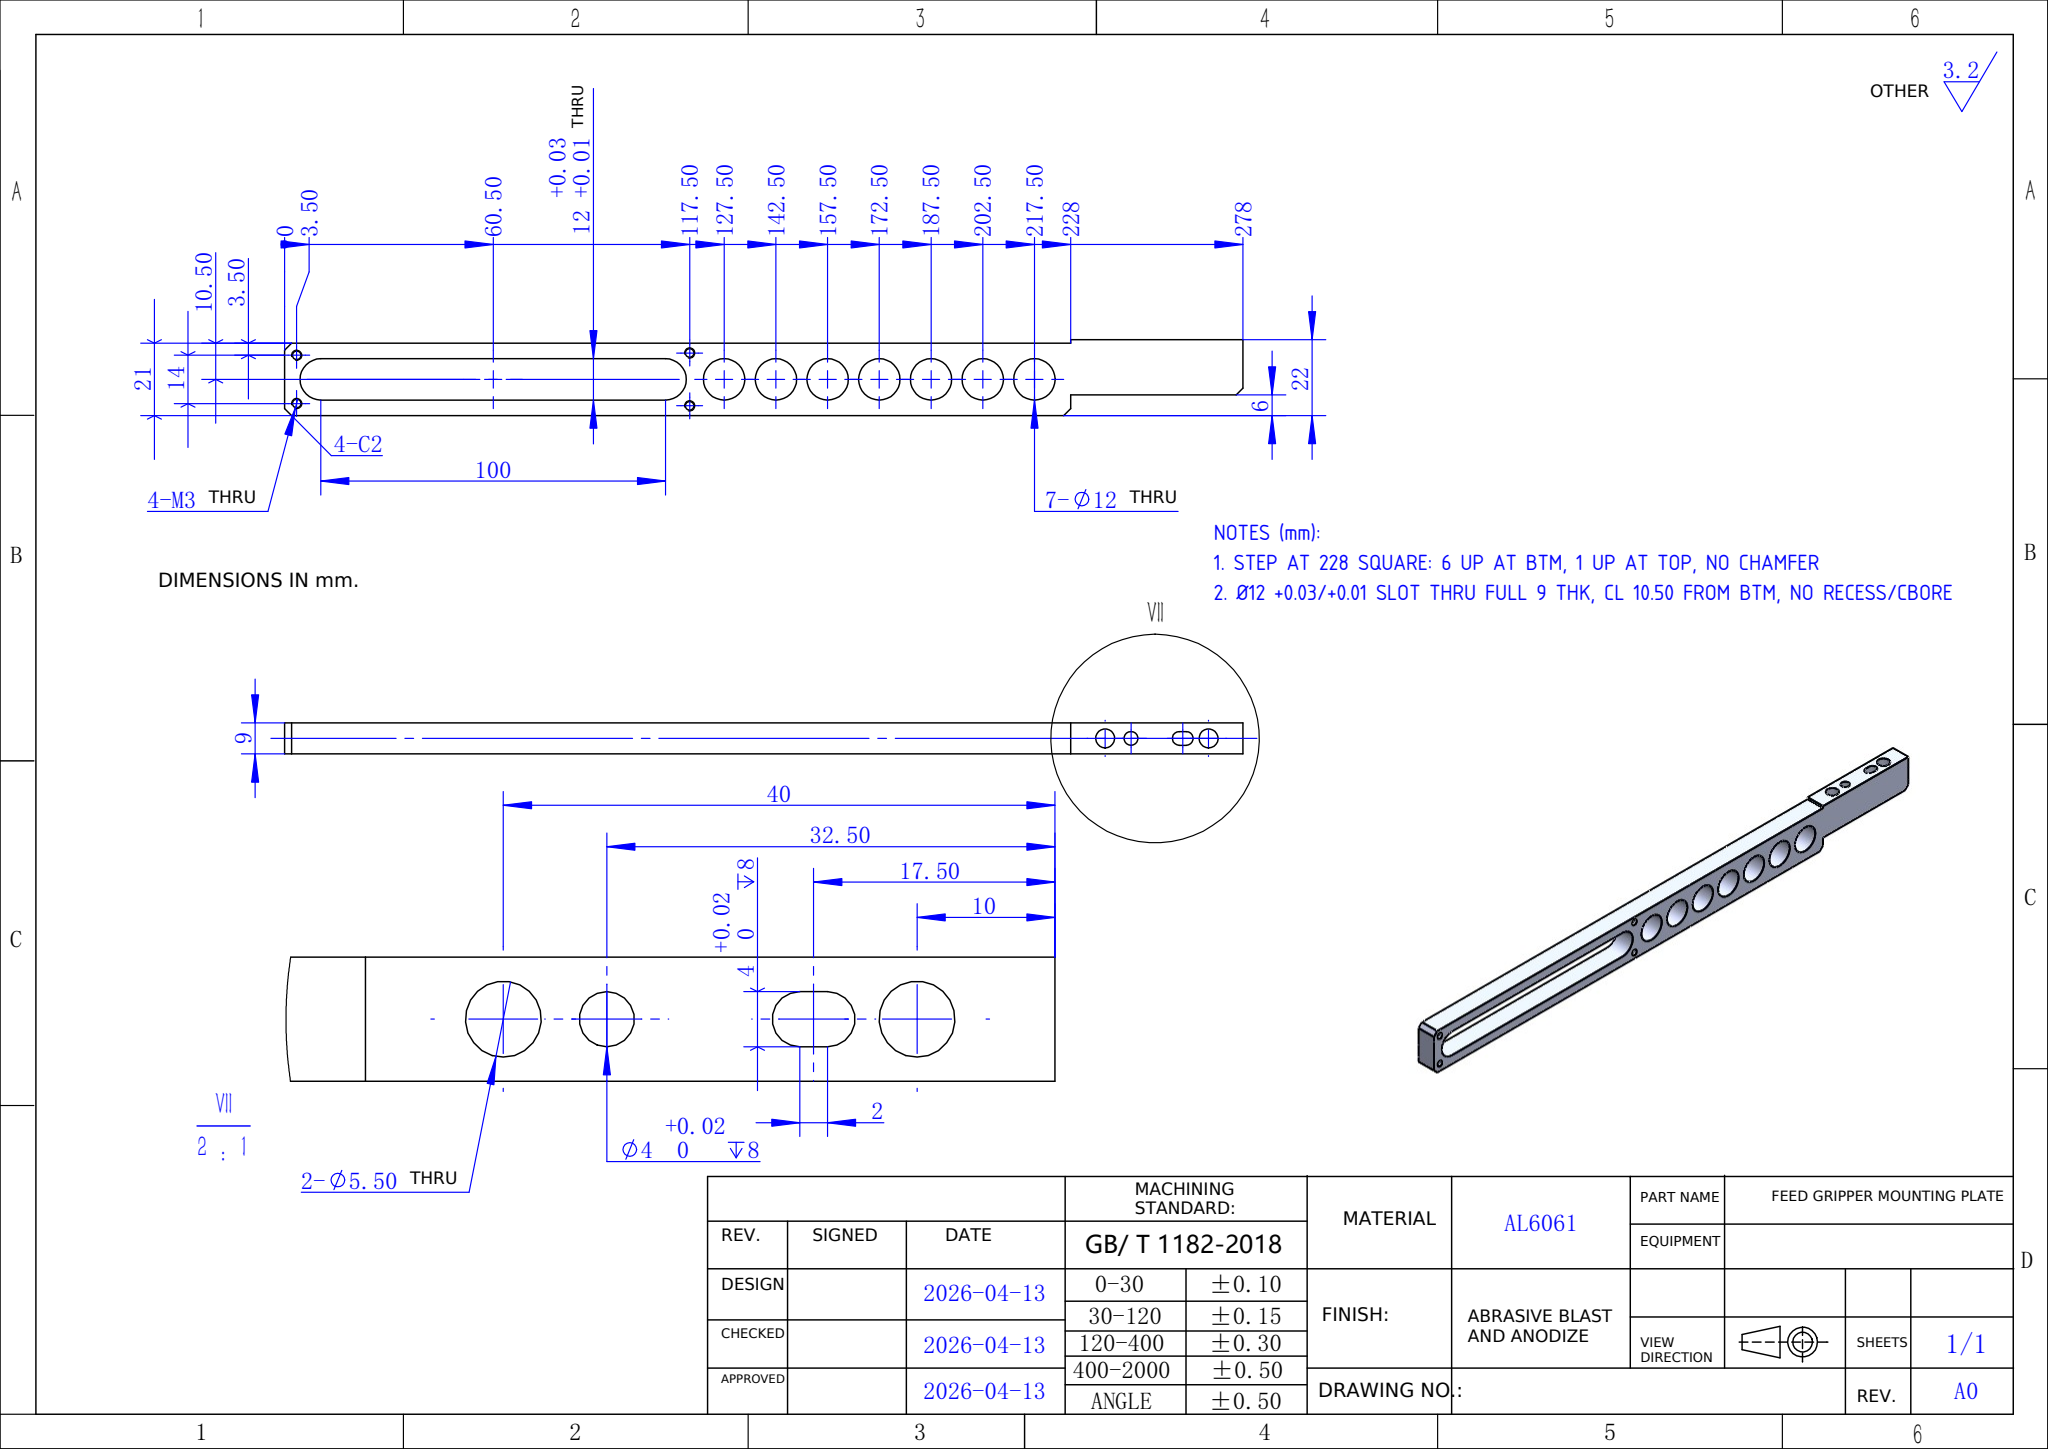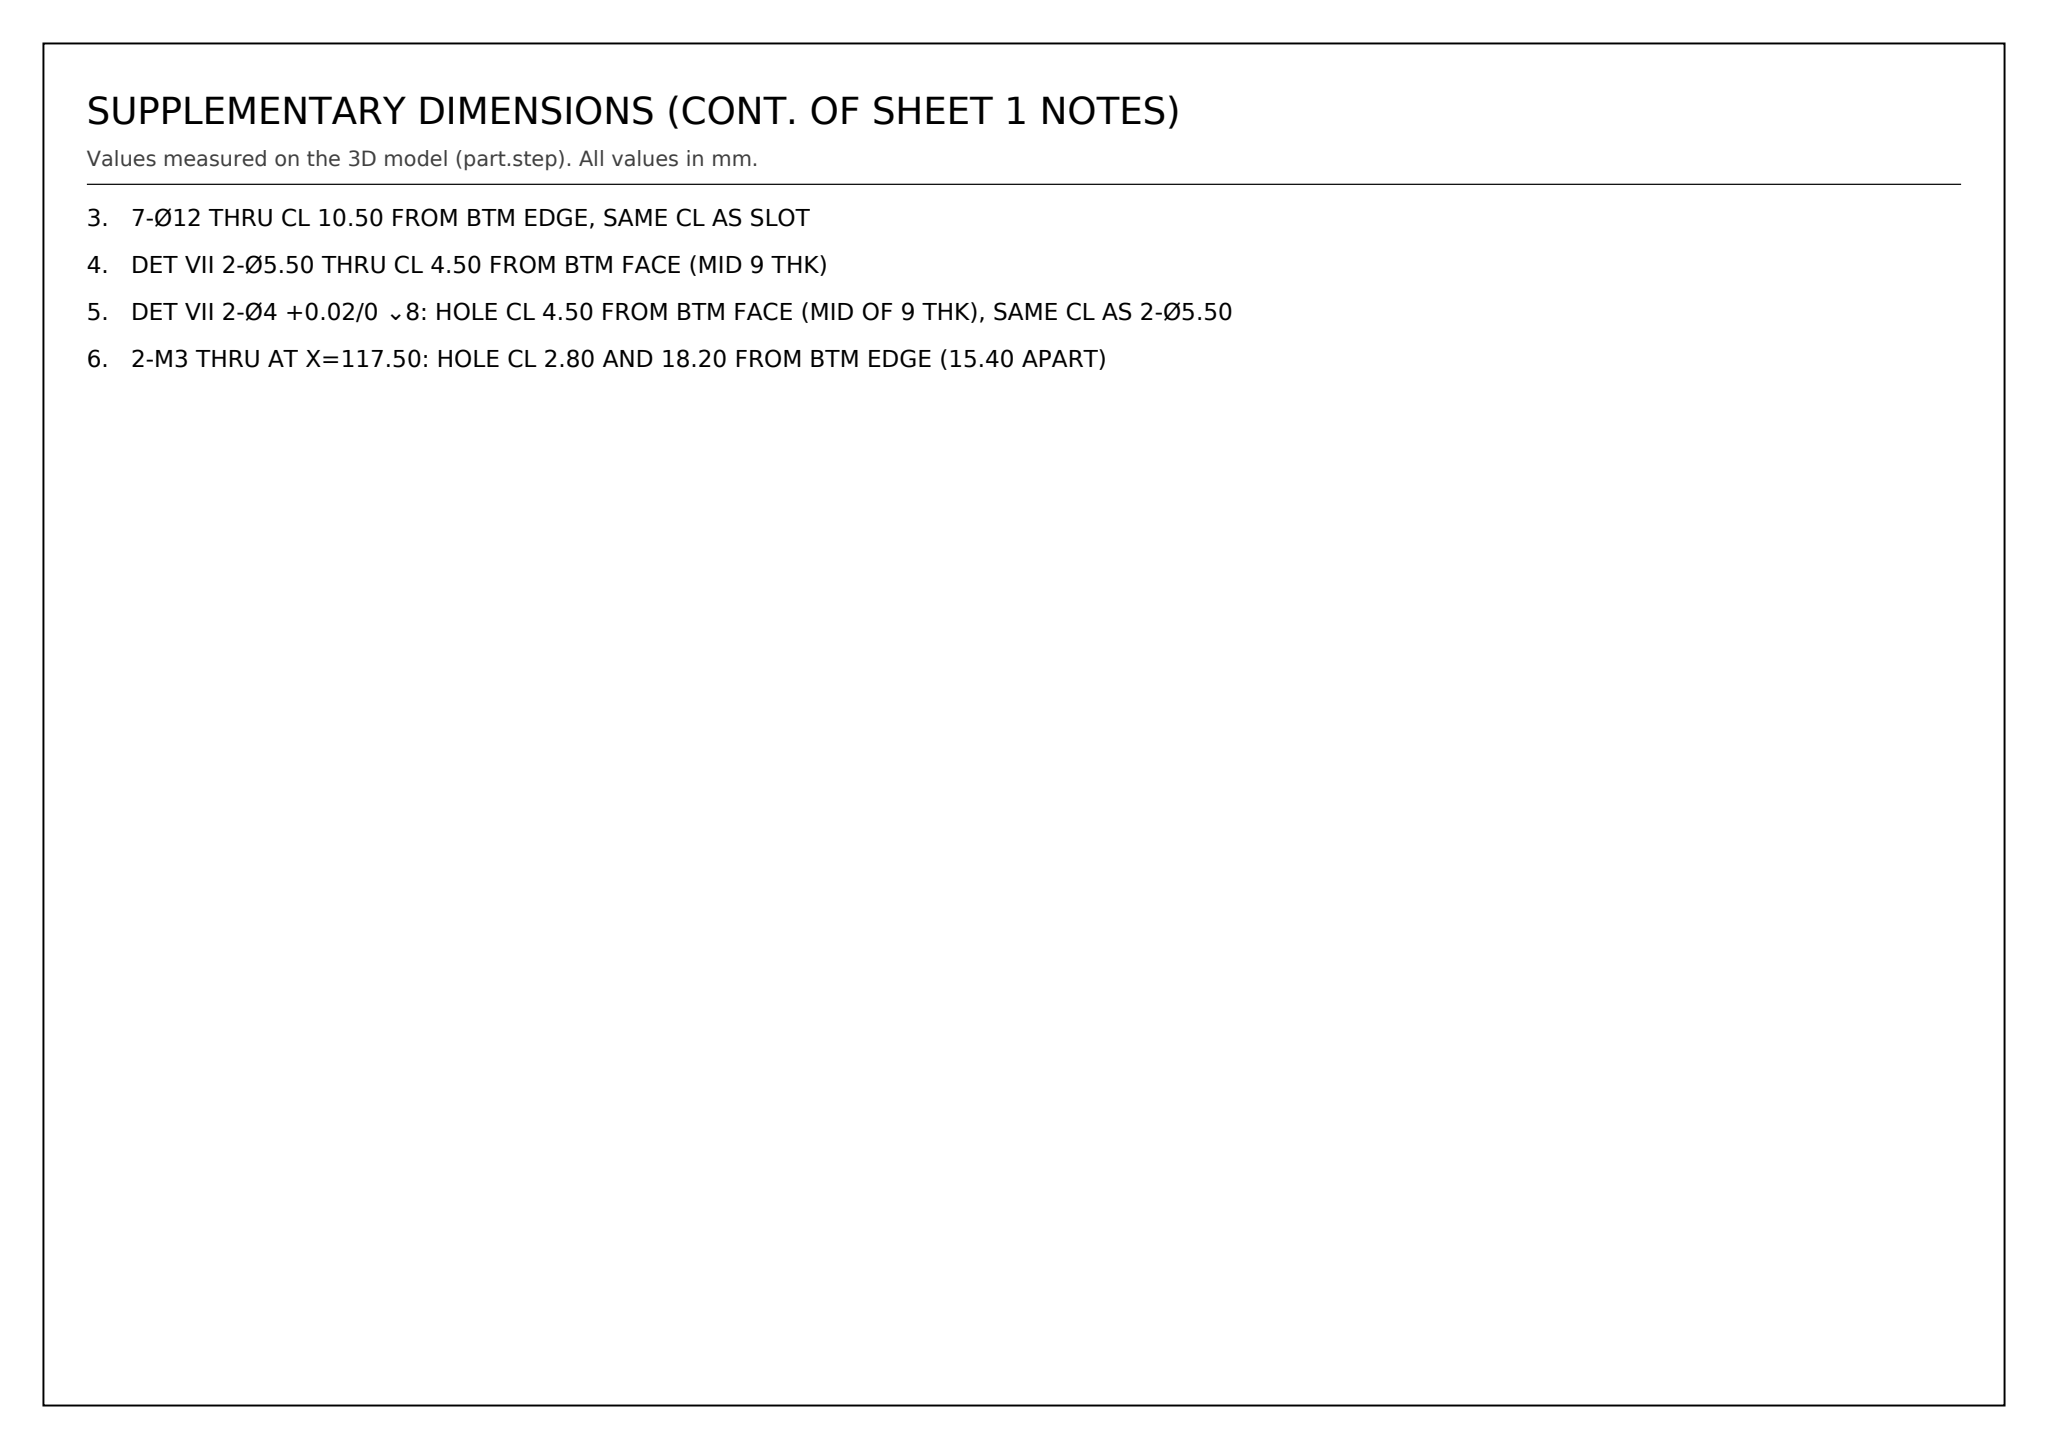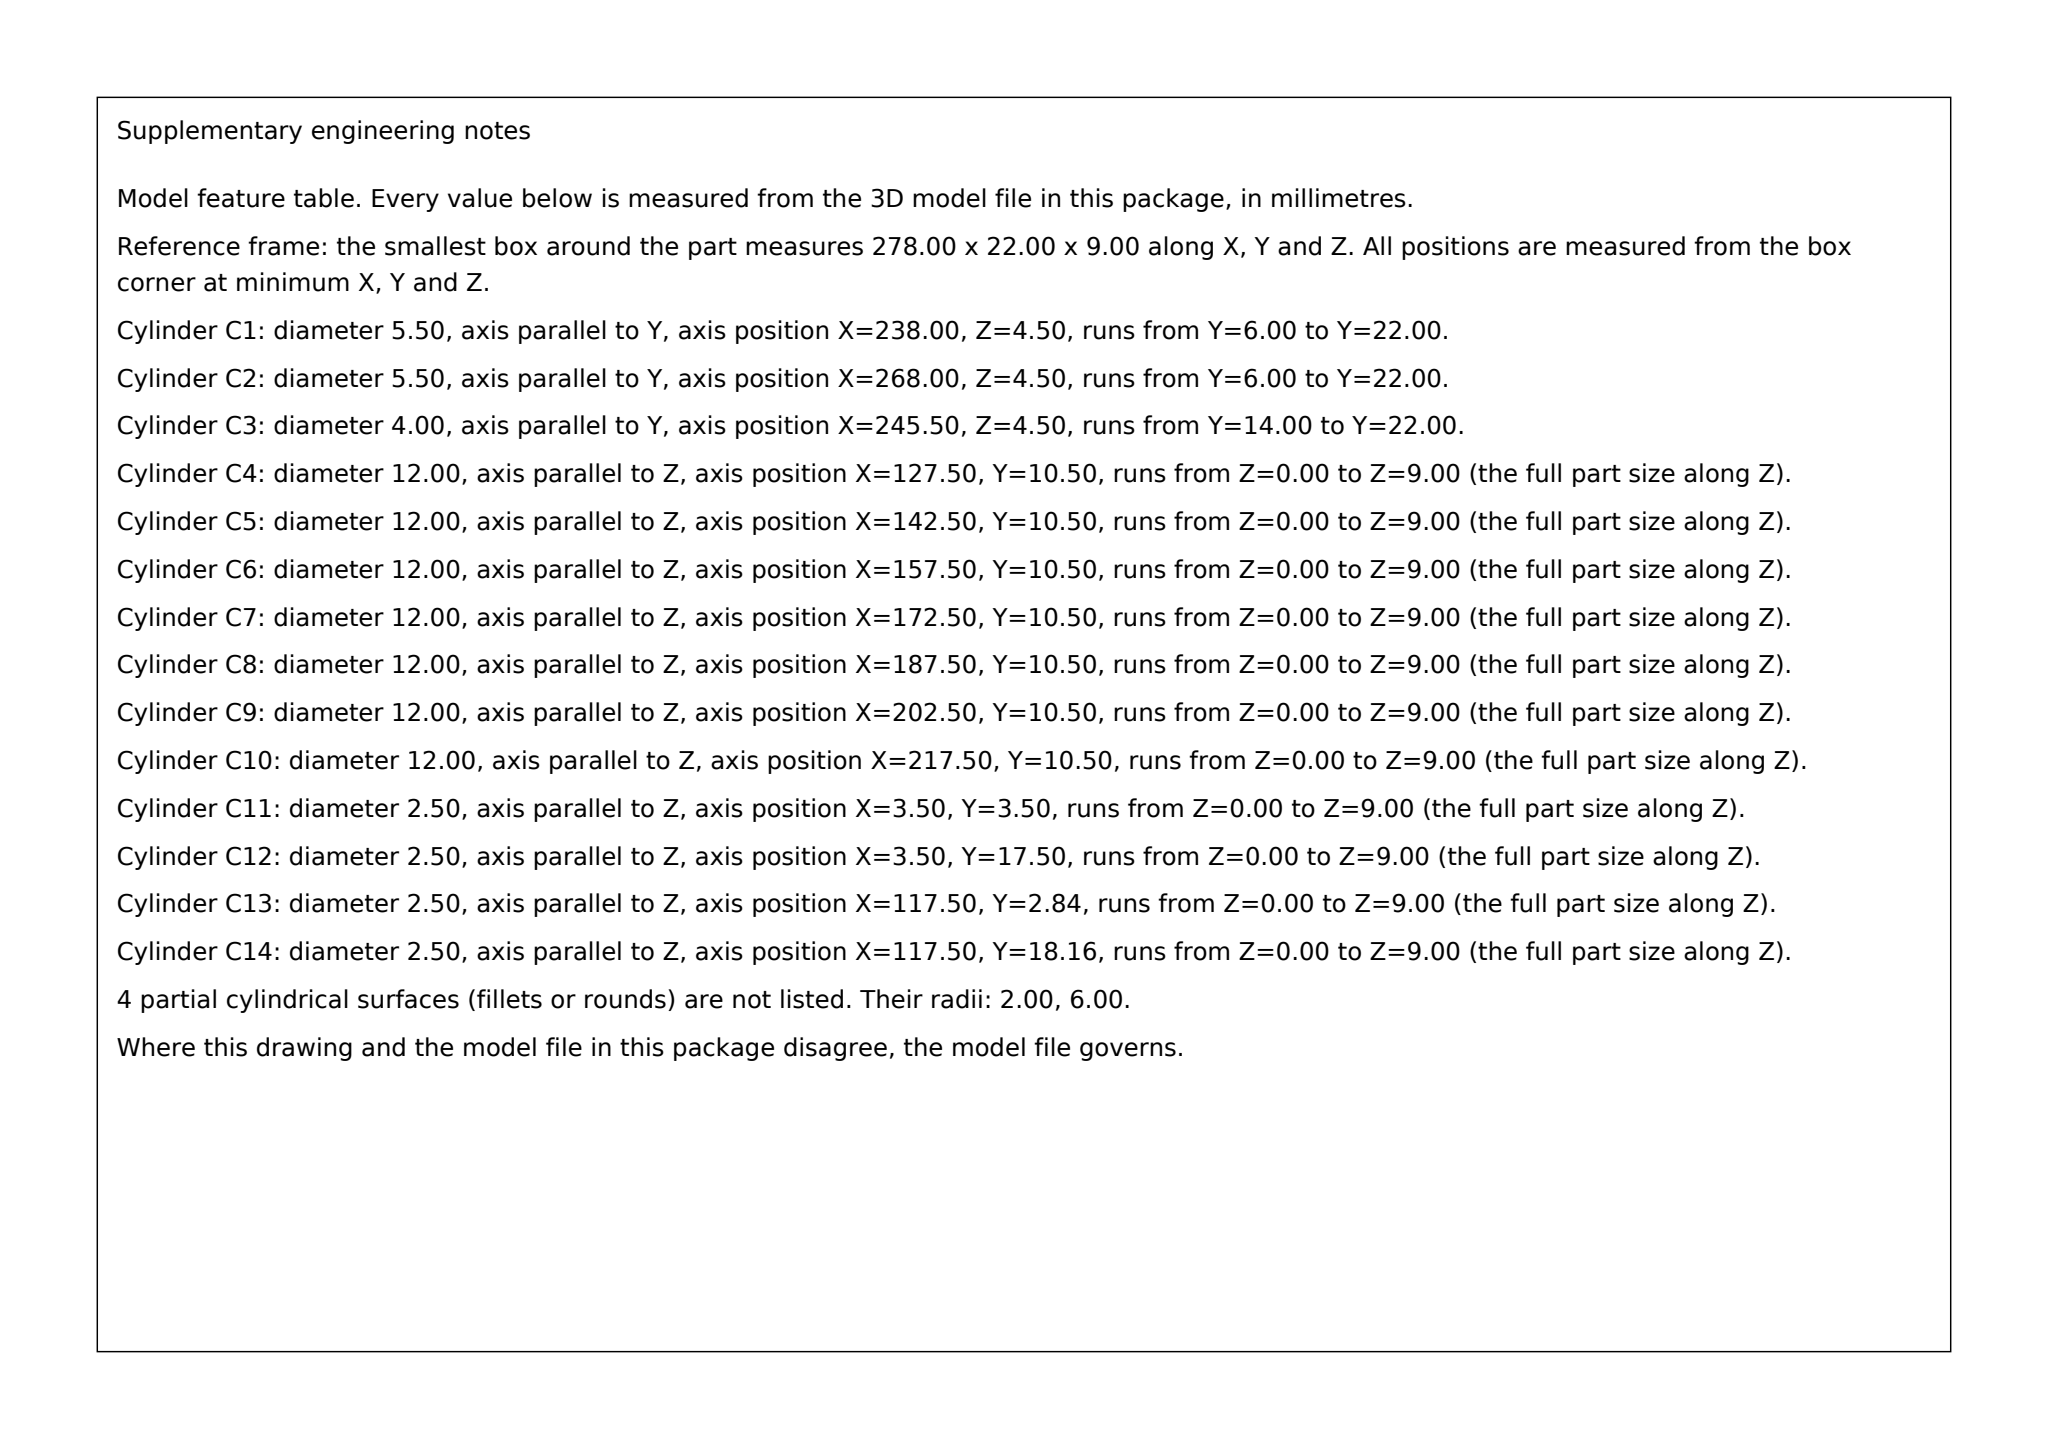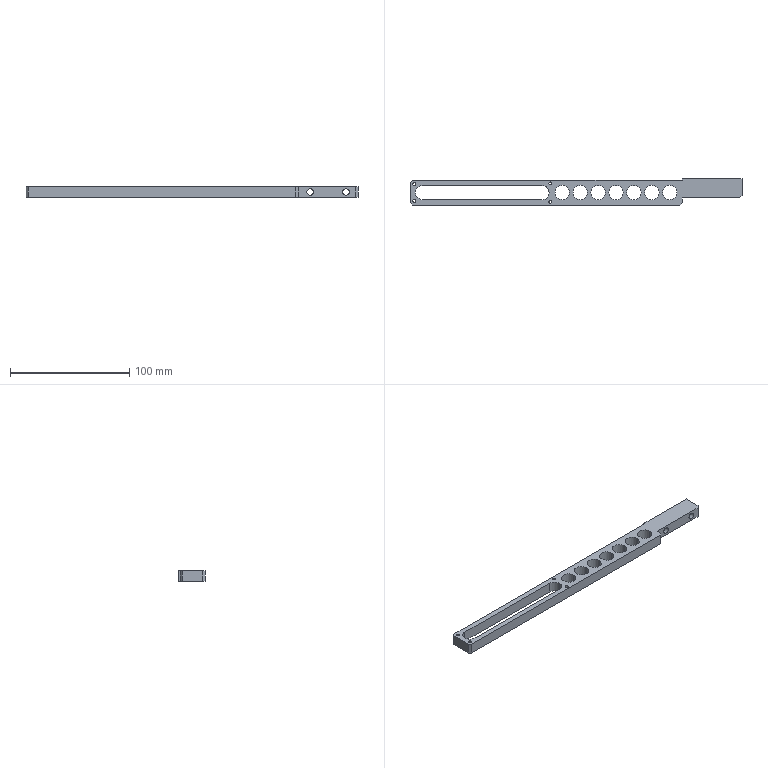Part | SolidWorks | mm | 1 solid | 53 faces | box 278 x 22 x 9 mm | volume 30075 mm3 | cylinder 33 | plane 20 | commonest cylinder face diameters 12 x17 2.5 x8 4 x4 5.5 x4
Drawing notes:
STEP AT 228 SQUARE: 6 UP AT BTM, 1 UP AT TOP, NO CHAMFER | from the solid: x-planes at 228 both normal to X; y-planes 0 & 6 (6 step btm), 21 & 22 (1 step top); no cone/angled face
Ø12 +0.03/+0.01 SLOT THRU FULL 9 THK, CL 10.50 FROM BTM, NO RECESS/CBORE | from the solid: Ø12 z-axis cyls at (10.5,10.5) & (110.5,10.5), length 9 = full thk; only y-planes 4.5 & 16.5 bound slot
7-Ø12 THRU CL 10.50 FROM BTM EDGE, SAME CL AS SLOT | from the solid: Ø12 z-axis holes at x=127.5...217.5, all y=10.5
DET VII 2-Ø5.50 THRU CL 4.50 FROM BTM FACE (MID 9 THK) | from the solid: Ø5.5 y-axis cylinders at z=4.5, x=238.0 & 268.0, length 16
DET VII 2-Ø4 +0.02/0 ⌄8: HOLE CL 4.50 FROM BTM FACE (MID OF 9 THK), SAME CL AS 2-Ø5.50 | from the solid: cylinders dia 4.0 axis y at axis_pos (245.5, -, 4.5) and arc pair at (259.5/261.5, -, 4.5), from y=14.0 to y=22.0 (8 deep); bbox z = 9.0
2-M3 THRU AT X=117.50: HOLE CL 2.80 AND 18.20 FROM BTM EDGE (15.40 APART) | from the solid: cylinders: hole/bore dia 2.5 axis z at [117.5, 18.2] and [117.5, 2.8], from z=0 to z=9 (THRU)
build123d program:
from build123d import *

# Parameters (mm, degrees)
BOSS_EXTRUDE1_DEPTH = 4.5
CHAMFER1_SIZE       = 2
CUT_EXTRUDE1_DEPTH  = 9
M3_TAPPED_HOLE1_D   = 2.5
SKETCH5_R           = 6
CUT_EXTRUDE2_DEPTH  = 9
SKETCH6_R           = 2.75
CUT_EXTRUDE3_DEPTH  = 279.905
SKETCH7_R           = 2
CUT_EXTRUDE4_DEPTH  = 8


with BuildPart() as part:
    # Sketch1 → Boss-Extrude1 (new, symmetric)
    with BuildSketch(Plane.XY):
        Polygon((0, 21), (0, 0), (228, 0), (228, 6), (278, 6), (278, 20.989), (278, 22), (228, 22), (228, 21), align=None)
    extrude(amount=BOSS_EXTRUDE1_DEPTH, both=True)

    # Chamfer1
    chamfer1_edges = [part.edges().sort_by_distance(p)[0] for p in [
        (278, 6, 0),
        (228, 0, 0),
        (0, 0, 0),
        (0, 21, 0),
    ]]
    chamfer(chamfer1_edges, length=CHAMFER1_SIZE)

    # Sketch2 → Cut-Extrude1 (cut)
    with BuildSketch(Plane.XY.offset(4.5)):
        with BuildLine():
            Line((10.5, 16.5), (110.5, 16.5))
            ThreePointArc((110.5, 16.5), (116.5, 10.5), (110.5, 4.5))
            Line((110.5, 4.5), (10.5, 4.5))
            ThreePointArc((10.5, 4.5), (4.5, 10.5), (10.5, 16.5))
        make_face()
    extrude(amount=-CUT_EXTRUDE1_DEPTH, mode=Mode.SUBTRACT)

    # M3 Tapped Hole1 (through all)
    with Locations(Plane.XY.offset(4.5)):
        with Locations((3.5, 17.5), (117.5, 18.161), (117.5, 2.839), (3.5, 3.5)):
            Hole(M3_TAPPED_HOLE1_D / 2)

    # Sketch5 → Cut-Extrude2 (cut)
    with BuildSketch(Plane.XY.offset(4.5)):
        with Locations((217.5, 10.5)):
            Circle(SKETCH5_R)
        with Locations((202.5, 10.5)):
            Circle(SKETCH5_R)
        with Locations((187.5, 10.5)):
            Circle(SKETCH5_R)
        with Locations((172.5, 10.5)):
            Circle(SKETCH5_R)
        with Locations((157.5, 10.5)):
            Circle(SKETCH5_R)
        with Locations((142.5, 10.5)):
            Circle(SKETCH5_R)
        with Locations((127.5, 10.5)):
            Circle(SKETCH5_R)
    extrude(amount=-CUT_EXTRUDE2_DEPTH, mode=Mode.SUBTRACT)

    # Sketch6 → Cut-Extrude3 (cut, through all)
    with BuildSketch(Plane(origin=(0, 22, 0), x_dir=(1, 0, 0), z_dir=(0, 1, 0))):
        with Locations(Location((268, 0, 0), (0, 0, 270))):
            Circle(SKETCH6_R)
        with Locations(Location((238, 0, 0), (0, 0, 270))):
            Circle(SKETCH6_R)
    extrude(amount=-CUT_EXTRUDE3_DEPTH, mode=Mode.SUBTRACT)

    # Sketch7 → Cut-Extrude4 (cut)
    with BuildSketch(Plane(origin=(0, 22, 0), x_dir=(1, 0, 0), z_dir=(0, 1, 0))):
        with Locations(Location((245.5, 0, 0), (0, 0, 270))):
            Circle(SKETCH7_R)
        with BuildLine():
            Line((259.5, 2), (261.5, 2))
            ThreePointArc((261.5, 2), (263.5, 0), (261.5, -2))
            Line((261.5, -2), (259.5, -2))
            ThreePointArc((259.5, -2), (257.5, 0), (259.5, 2))
        make_face()
    extrude(amount=-CUT_EXTRUDE4_DEPTH, mode=Mode.SUBTRACT)


solid = part.part